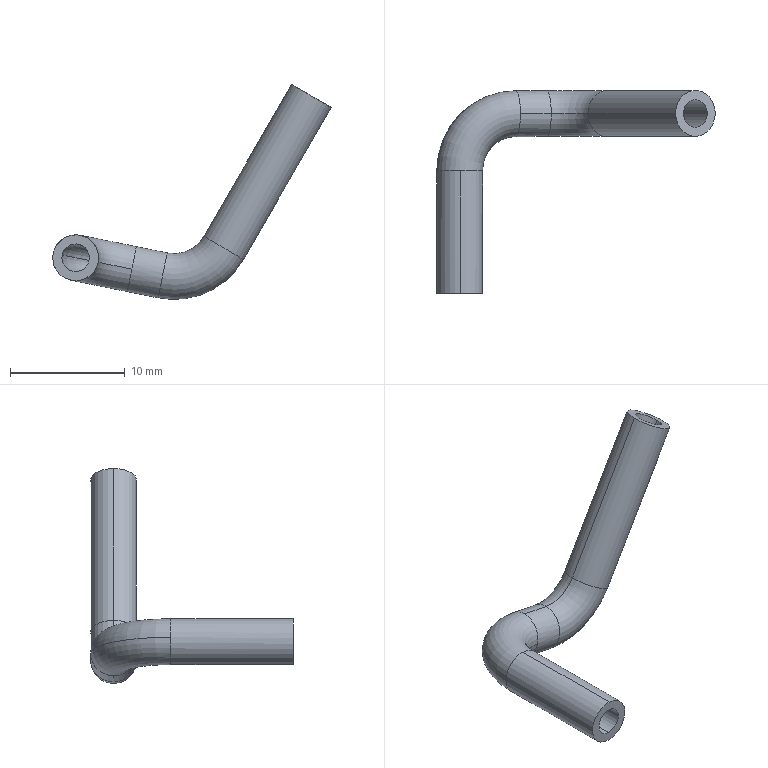Component | SolidWorks | WaterPipe7-1 | 1 solid | 22 faces | box 24.3 x 17.68 x 18.75 mm | volume 344 mm3 | cylinder 12 | torus 8 | plane 2 | commonest cylinder face diameters 2.4 x6 4 x6
build123d program:
from build123d import *

# Parameters (mm, degrees)
SCAN_THIN_FEATURE1_PROFILE_R   = 2
SCAN_THIN_FEATURE1_PROFILE_R_2 = 1.2


with BuildPart() as part:
    # Scan-Thin Feature1: sweep along a curve in space
    with BuildLine() as scan_thin_feature1_path:
        Line((10, -15, 0), (10, -4.322, 0))
        ThreePointArc((5.069, 0.6783, 0.8273), (8.556, -0.7862, 0.2423), (10, -4.322, 0))
        Line((5.069, 0.6783, 0.8273), (2.362, 0.6783, 1.281))
        ThreePointArc((-2.879, 0.6783, -1.299), (-0.6744, 0.6783, 0.836), (2.362, 0.6783, 1.281))
        Line((-2.879, 0.6783, -1.299), (-10.072, 0.6783, -14.805))
    # Scan-Thin Feature1 profile (on start of the path) → Scan-Thin Feature1 (sweep)
    with BuildSketch(Plane(origin=(10, -15, 0), x_dir=(0, 0, 1), z_dir=(0, 1, 0))):
        Circle(SCAN_THIN_FEATURE1_PROFILE_R)
        Circle(SCAN_THIN_FEATURE1_PROFILE_R_2, mode=Mode.SUBTRACT)
    sweep(path=scan_thin_feature1_path.line)


solid = part.part

# Placed as in the assembly
solid = solid.moved(Location((14.013, 32.882, 79.658), (180, -1.96, -180)))
STEP:
#1=COLOUR_RGB('',0.7922,0.8196,0.9333);
#2=FILL_AREA_STYLE_COLOUR('',#1);
#3=FILL_AREA_STYLE('',(#2));
#4=SURFACE_STYLE_FILL_AREA(#3);
#5=SURFACE_SIDE_STYLE('',(#4));
#6=SURFACE_STYLE_USAGE(.BOTH.,#5);
#7=PRESENTATION_STYLE_ASSIGNMENT((#6));
#8=CARTESIAN_POINT('',(0.4665,1.321,3.135));
#9=VERTEX_POINT('',#8);
#10=CARTESIAN_POINT('',(0.4476,1.321,3.043));
#11=VERTEX_POINT('',#10);
#12=CARTESIAN_POINT('',(0.457,1.321,3.089));
#13=DIRECTION('',(-0.98,-0.,0.1991));
#14=DIRECTION('',(-0.1991,0.,-0.98));
#15=AXIS2_PLACEMENT_3D('',#12,#13,#14);
#16=CIRCLE('',#15,0.04724);
#17=EDGE_CURVE('',#9,#11,#16,.T.);
#18=ORIENTED_EDGE('',*,*,#17,.T.);
#19=CARTESIAN_POINT('',(0.7076,1.321,3.16));
#20=VERTEX_POINT('',#19);
#21=CARTESIAN_POINT('',(0.4962,1.321,3.282));
#22=DIRECTION('',(0.,-1.,0.));
#23=DIRECTION('',(0.,0.,-1.));
#24=AXIS2_PLACEMENT_3D('',#21,#22,#23);
#25=CIRCLE('',#24,0.2441);
#26=EDGE_CURVE('',#11,#20,#25,.T.);
#27=ORIENTED_EDGE('',*,*,#26,.T.);
#28=CARTESIAN_POINT('',(0.6258,1.321,3.207));
#29=VERTEX_POINT('',#28);
#30=CARTESIAN_POINT('',(0.6667,1.321,3.183));
#31=DIRECTION('',(-0.5,-0.,-0.866));
#32=DIRECTION('',(-0.866,0.,0.5));
#33=AXIS2_PLACEMENT_3D('',#30,#31,#32);
#34=CIRCLE('',#33,0.04724);
#35=EDGE_CURVE('',#29,#20,#34,.T.);
#36=ORIENTED_EDGE('',*,*,#35,.F.);
#37=CARTESIAN_POINT('',(0.4962,1.321,3.282));
#38=DIRECTION('',(0.,-1.,0.));
#39=DIRECTION('',(0.,0.,-1.));
#40=AXIS2_PLACEMENT_3D('',#37,#38,#39);
#41=CIRCLE('',#40,0.1496);
#42=EDGE_CURVE('',#9,#29,#41,.T.);
#43=ORIENTED_EDGE('',*,*,#42,.F.);
#44=EDGE_LOOP('',(#18,#27,#36,#43));
#45=FACE_OUTER_BOUND('',#44,.T.);
#46=CARTESIAN_POINT('',(0.4962,1.321,3.282));
#47=DIRECTION('',(0.,-1.,0.));
#48=DIRECTION('',(0.03421,0.,0.9994));
#49=AXIS2_PLACEMENT_3D('',#46,#47,#48);
#50=TOROIDAL_SURFACE('',#49,0.1969,0.04724);
#51=ADVANCED_FACE('',(#45),#50,.F.);
#52=CARTESIAN_POINT('',(0.1598,1.124,3.197));
#53=VERTEX_POINT('',#52);
#54=CARTESIAN_POINT('',(0.1119,1.124,3.159));
#55=VERTEX_POINT('',#54);
#56=CARTESIAN_POINT('',(0.1582,1.124,3.15));
#57=DIRECTION('',(0.,-1.,0.));
#58=DIRECTION('',(-0.03421,0.,-0.9994));
#59=AXIS2_PLACEMENT_3D('',#56,#57,#58);
#60=CIRCLE('',#59,0.04724);
#61=EDGE_CURVE('',#53,#55,#60,.T.);
#62=ORIENTED_EDGE('',*,*,#61,.T.);
#63=CARTESIAN_POINT('',(0.3511,1.369,3.11));
#64=VERTEX_POINT('',#63);
#65=CARTESIAN_POINT('',(0.3511,1.124,3.11));
#66=DIRECTION('',(-0.1991,-0.,-0.98));
#67=DIRECTION('',(-0.98,0.,0.1991));
#68=AXIS2_PLACEMENT_3D('',#65,#66,#67);
#69=CIRCLE('',#68,0.2441);
#70=EDGE_CURVE('',#55,#64,#69,.T.);
#71=ORIENTED_EDGE('',*,*,#70,.T.);
#72=CARTESIAN_POINT('',(0.3605,1.321,3.157));
#73=VERTEX_POINT('',#72);
#74=CARTESIAN_POINT('',(0.3511,1.321,3.11));
#75=DIRECTION('',(-0.98,-0.,0.1991));
#76=DIRECTION('',(0.1991,0.,0.98));
#77=AXIS2_PLACEMENT_3D('',#74,#75,#76);
#78=CIRCLE('',#77,0.04724);
#79=EDGE_CURVE('',#73,#64,#78,.T.);
#80=ORIENTED_EDGE('',*,*,#79,.F.);
#81=CARTESIAN_POINT('',(0.3511,1.274,3.11));
#82=VERTEX_POINT('',#81);
#83=CARTESIAN_POINT('',(0.3511,1.321,3.11));
#84=DIRECTION('',(-0.98,-0.,0.1991));
#85=DIRECTION('',(0.1991,0.,0.98));
#86=AXIS2_PLACEMENT_3D('',#83,#84,#85);
#87=CIRCLE('',#86,0.04724);
#88=EDGE_CURVE('',#82,#73,#87,.T.);
#89=ORIENTED_EDGE('',*,*,#88,.F.);
#90=CARTESIAN_POINT('',(0.2045,1.124,3.14));
#91=VERTEX_POINT('',#90);
#92=CARTESIAN_POINT('',(0.3511,1.124,3.11));
#93=DIRECTION('',(-0.1991,-0.,-0.98));
#94=DIRECTION('',(-0.98,0.,0.1991));
#95=AXIS2_PLACEMENT_3D('',#92,#93,#94);
#96=CIRCLE('',#95,0.1496);
#97=EDGE_CURVE('',#91,#82,#96,.T.);
#98=ORIENTED_EDGE('',*,*,#97,.F.);
#99=CARTESIAN_POINT('',(0.1582,1.124,3.15));
#100=DIRECTION('',(0.,-1.,0.));
#101=DIRECTION('',(-0.03421,0.,-0.9994));
#102=AXIS2_PLACEMENT_3D('',#99,#100,#101);
#103=CIRCLE('',#102,0.04724);
#104=EDGE_CURVE('',#91,#53,#103,.T.);
#105=ORIENTED_EDGE('',*,*,#104,.T.);
#106=EDGE_LOOP('',(#62,#71,#80,#89,#98,#105));
#107=FACE_OUTER_BOUND('',#106,.T.);
#108=CARTESIAN_POINT('',(0.3511,1.124,3.11));
#109=DIRECTION('',(-0.1991,-0.,-0.98));
#110=DIRECTION('',(-0.98,-0.,0.1991));
#111=AXIS2_PLACEMENT_3D('',#108,#109,#110);
#112=TOROIDAL_SURFACE('',#111,0.1969,0.04724);
#113=ADVANCED_FACE('',(#107),#112,.F.);
#114=CARTESIAN_POINT('',(0.4414,1.321,3.012));
#115=VERTEX_POINT('',#114);
#116=CARTESIAN_POINT('',(0.4727,1.321,3.166));
#117=VERTEX_POINT('',#116);
#118=CARTESIAN_POINT('',(0.457,1.321,3.089));
#119=DIRECTION('',(-0.98,-0.,0.1991));
#120=DIRECTION('',(0.1991,0.,0.98));
#121=AXIS2_PLACEMENT_3D('',#118,#119,#120);
#122=CIRCLE('',#121,0.07874);
#123=EDGE_CURVE('',#115,#117,#122,.T.);
#124=ORIENTED_EDGE('',*,*,#123,.F.);
#125=CARTESIAN_POINT('',(0.7349,1.321,3.144));
#126=VERTEX_POINT('',#125);
#127=CARTESIAN_POINT('',(0.4962,1.321,3.282));
#128=DIRECTION('',(0.,-1.,0.));
#129=DIRECTION('',(0.,0.,-1.));
#130=AXIS2_PLACEMENT_3D('',#127,#128,#129);
#131=CIRCLE('',#130,0.2756);
#132=EDGE_CURVE('',#115,#126,#131,.T.);
#133=ORIENTED_EDGE('',*,*,#132,.T.);
#134=CARTESIAN_POINT('',(0.5985,1.321,3.223));
#135=VERTEX_POINT('',#134);
#136=CARTESIAN_POINT('',(0.6667,1.321,3.183));
#137=DIRECTION('',(-0.5,-0.,-0.866));
#138=DIRECTION('',(-0.866,0.,0.5));
#139=AXIS2_PLACEMENT_3D('',#136,#137,#138);
#140=CIRCLE('',#139,0.07874);
#141=EDGE_CURVE('',#126,#135,#140,.T.);
#142=ORIENTED_EDGE('',*,*,#141,.T.);
#143=CARTESIAN_POINT('',(0.4962,1.321,3.282));
#144=DIRECTION('',(0.,-1.,0.));
#145=DIRECTION('',(0.,0.,-1.));
#146=AXIS2_PLACEMENT_3D('',#143,#144,#145);
#147=CIRCLE('',#146,0.1181);
#148=EDGE_CURVE('',#117,#135,#147,.T.);
#149=ORIENTED_EDGE('',*,*,#148,.F.);
#150=EDGE_LOOP('',(#124,#133,#142,#149));
#151=FACE_OUTER_BOUND('',#150,.T.);
#152=CARTESIAN_POINT('',(0.4962,1.321,3.282));
#153=DIRECTION('',(0.,-1.,0.));
#154=DIRECTION('',(0.03421,0.,0.9994));
#155=AXIS2_PLACEMENT_3D('',#152,#153,#154);
#156=TOROIDAL_SURFACE('',#155,0.1969,0.07874);
#157=ADVANCED_FACE('',(#151),#156,.T.);
#158=CARTESIAN_POINT('',(0.08107,1.124,3.165));
#159=VERTEX_POINT('',#158);
#160=CARTESIAN_POINT('',(0.1555,1.124,3.071));
#161=VERTEX_POINT('',#160);
#162=CARTESIAN_POINT('',(0.1582,1.124,3.15));
#163=DIRECTION('',(0.,-1.,0.));
#164=DIRECTION('',(0.1991,0.,0.98));
#165=AXIS2_PLACEMENT_3D('',#162,#163,#164);
#166=CIRCLE('',#165,0.07874);
#167=EDGE_CURVE('',#159,#161,#166,.T.);
#168=ORIENTED_EDGE('',*,*,#167,.F.);
#169=CARTESIAN_POINT('',(0.3511,1.4,3.11));
#170=VERTEX_POINT('',#169);
#171=CARTESIAN_POINT('',(0.3511,1.124,3.11));
#172=DIRECTION('',(-0.1991,-0.,-0.98));
#173=DIRECTION('',(-0.98,0.,0.1991));
#174=AXIS2_PLACEMENT_3D('',#171,#172,#173);
#175=CIRCLE('',#174,0.2756);
#176=EDGE_CURVE('',#159,#170,#175,.T.);
#177=ORIENTED_EDGE('',*,*,#176,.T.);
#178=CARTESIAN_POINT('',(0.3355,1.321,3.033));
#179=VERTEX_POINT('',#178);
#180=CARTESIAN_POINT('',(0.3511,1.321,3.11));
#181=DIRECTION('',(-0.98,-0.,0.1991));
#182=DIRECTION('',(0.1991,0.,0.98));
#183=AXIS2_PLACEMENT_3D('',#180,#181,#182);
#184=CIRCLE('',#183,0.07874);
#185=EDGE_CURVE('',#170,#179,#184,.T.);
#186=ORIENTED_EDGE('',*,*,#185,.T.);
#187=CARTESIAN_POINT('',(0.3511,1.243,3.11));
#188=VERTEX_POINT('',#187);
#189=CARTESIAN_POINT('',(0.3511,1.321,3.11));
#190=DIRECTION('',(-0.98,-0.,0.1991));
#191=DIRECTION('',(0.1991,0.,0.98));
#192=AXIS2_PLACEMENT_3D('',#189,#190,#191);
#193=CIRCLE('',#192,0.07874);
#194=EDGE_CURVE('',#179,#188,#193,.T.);
#195=ORIENTED_EDGE('',*,*,#194,.T.);
#196=CARTESIAN_POINT('',(0.2354,1.124,3.134));
#197=VERTEX_POINT('',#196);
#198=CARTESIAN_POINT('',(0.3511,1.124,3.11));
#199=DIRECTION('',(-0.1991,-0.,-0.98));
#200=DIRECTION('',(-0.98,0.,0.1991));
#201=AXIS2_PLACEMENT_3D('',#198,#199,#200);
#202=CIRCLE('',#201,0.1181);
#203=EDGE_CURVE('',#197,#188,#202,.T.);
#204=ORIENTED_EDGE('',*,*,#203,.F.);
#205=CARTESIAN_POINT('',(0.1582,1.124,3.15));
#206=DIRECTION('',(0.,-1.,0.));
#207=DIRECTION('',(0.1991,0.,0.98));
#208=AXIS2_PLACEMENT_3D('',#205,#206,#207);
#209=CIRCLE('',#208,0.07874);
#210=EDGE_CURVE('',#161,#197,#209,.T.);
#211=ORIENTED_EDGE('',*,*,#210,.F.);
#212=EDGE_LOOP('',(#168,#177,#186,#195,#204,#211));
#213=FACE_OUTER_BOUND('',#212,.T.);
#214=CARTESIAN_POINT('',(0.3511,1.124,3.11));
#215=DIRECTION('',(-0.1991,-0.,-0.98));
#216=DIRECTION('',(-0.98,0.,0.1991));
#217=AXIS2_PLACEMENT_3D('',#214,#215,#216);
#218=TOROIDAL_SURFACE('',#217,0.1969,0.07874);
#219=ADVANCED_FACE('',(#213),#218,.T.);
#220=CARTESIAN_POINT('',(0.6667,1.321,3.183));
#221=DIRECTION('',(-0.5,-0.,-0.866));
#222=DIRECTION('',(-0.866,0.,0.5));
#223=AXIS2_PLACEMENT_3D('',#220,#221,#222);
#224=CIRCLE('',#223,0.04724);
#225=EDGE_CURVE('',#20,#29,#224,.T.);
#226=ORIENTED_EDGE('',*,*,#225,.T.);
#227=CARTESIAN_POINT('',(0.927,1.321,3.729));
#228=VERTEX_POINT('',#227);
#229=CARTESIAN_POINT('',(0.6258,1.321,3.207));
#230=DIRECTION('',(0.5,0.,0.866));
#231=VECTOR('',#230,39.37);
#232=LINE('',#229,#231);
#233=EDGE_CURVE('',#29,#228,#232,.T.);
#234=ORIENTED_EDGE('',*,*,#233,.T.);
#235=CARTESIAN_POINT('',(1.009,1.321,3.681));
#236=VERTEX_POINT('',#235);
#237=CARTESIAN_POINT('',(0.9679,1.321,3.705));
#238=DIRECTION('',(-0.5,-0.,-0.866));
#239=DIRECTION('',(-0.866,0.,0.5));
#240=AXIS2_PLACEMENT_3D('',#237,#238,#239);
#241=CIRCLE('',#240,0.04724);
#242=EDGE_CURVE('',#236,#228,#241,.T.);
#243=ORIENTED_EDGE('',*,*,#242,.F.);
#244=CARTESIAN_POINT('',(0.7076,1.321,3.16));
#245=DIRECTION('',(0.5,0.,0.866));
#246=VECTOR('',#245,39.37);
#247=LINE('',#244,#246);
#248=EDGE_CURVE('',#20,#236,#247,.T.);
#249=ORIENTED_EDGE('',*,*,#248,.F.);
#250=EDGE_LOOP('',(#226,#234,#243,#249));
#251=FACE_OUTER_BOUND('',#250,.T.);
#252=CARTESIAN_POINT('',(0.6667,1.321,3.183));
#253=DIRECTION('',(0.5,0.,0.866));
#254=DIRECTION('',(0.866,0.,-0.5));
#255=AXIS2_PLACEMENT_3D('',#252,#253,#254);
#256=CYLINDRICAL_SURFACE('',#255,0.04724);
#257=ADVANCED_FACE('',(#251),#256,.F.);
#258=CARTESIAN_POINT('',(0.3417,1.321,3.064));
#259=VERTEX_POINT('',#258);
#260=CARTESIAN_POINT('',(0.3511,1.321,3.11));
#261=DIRECTION('',(-0.98,-0.,0.1991));
#262=DIRECTION('',(0.1991,0.,0.98));
#263=AXIS2_PLACEMENT_3D('',#260,#261,#262);
#264=CIRCLE('',#263,0.04724);
#265=EDGE_CURVE('',#259,#82,#264,.T.);
#266=ORIENTED_EDGE('',*,*,#265,.T.);
#267=ORIENTED_EDGE('',*,*,#88,.T.);
#268=CARTESIAN_POINT('',(0.3605,1.321,3.157));
#269=DIRECTION('',(0.98,0.,-0.1991));
#270=VECTOR('',#269,39.37);
#271=LINE('',#268,#270);
#272=EDGE_CURVE('',#73,#9,#271,.T.);
#273=ORIENTED_EDGE('',*,*,#272,.T.);
#274=CARTESIAN_POINT('',(0.457,1.321,3.089));
#275=DIRECTION('',(-0.98,-0.,0.1991));
#276=DIRECTION('',(-0.1991,0.,-0.98));
#277=AXIS2_PLACEMENT_3D('',#274,#275,#276);
#278=CIRCLE('',#277,0.04724);
#279=EDGE_CURVE('',#11,#9,#278,.T.);
#280=ORIENTED_EDGE('',*,*,#279,.F.);
#281=CARTESIAN_POINT('',(0.3417,1.321,3.064));
#282=DIRECTION('',(0.98,0.,-0.1991));
#283=VECTOR('',#282,39.37);
#284=LINE('',#281,#283);
#285=EDGE_CURVE('',#259,#11,#284,.T.);
#286=ORIENTED_EDGE('',*,*,#285,.F.);
#287=EDGE_LOOP('',(#266,#267,#273,#280,#286));
#288=FACE_OUTER_BOUND('',#287,.T.);
#289=CARTESIAN_POINT('',(0.3511,1.321,3.11));
#290=DIRECTION('',(0.98,0.,-0.1991));
#291=DIRECTION('',(-0.1991,0.,-0.98));
#292=AXIS2_PLACEMENT_3D('',#289,#290,#291);
#293=CYLINDRICAL_SURFACE('',#292,0.04724);
#294=ADVANCED_FACE('',(#288),#293,.F.);
#295=CARTESIAN_POINT('',(0.1566,0.704,3.102));
#296=VERTEX_POINT('',#295);
#297=CARTESIAN_POINT('',(0.1598,0.704,3.197));
#298=VERTEX_POINT('',#297);
#299=CARTESIAN_POINT('',(0.1582,0.704,3.15));
#300=DIRECTION('',(0.,-1.,0.));
#301=DIRECTION('',(0.03421,0.,0.9994));
#302=AXIS2_PLACEMENT_3D('',#299,#300,#301);
#303=CIRCLE('',#302,0.04724);
#304=EDGE_CURVE('',#296,#298,#303,.T.);
#305=ORIENTED_EDGE('',*,*,#304,.T.);
#306=CARTESIAN_POINT('',(0.1598,0.704,3.197));
#307=DIRECTION('',(-0.,1.,-0.));
#308=VECTOR('',#307,39.37);
#309=LINE('',#306,#308);
#310=EDGE_CURVE('',#298,#53,#309,.T.);
#311=ORIENTED_EDGE('',*,*,#310,.T.);
#312=ORIENTED_EDGE('',*,*,#104,.F.);
#313=CARTESIAN_POINT('',(0.1566,1.124,3.102));
#314=VERTEX_POINT('',#313);
#315=CARTESIAN_POINT('',(0.1582,1.124,3.15));
#316=DIRECTION('',(0.,-1.,0.));
#317=DIRECTION('',(-0.03421,0.,-0.9994));
#318=AXIS2_PLACEMENT_3D('',#315,#316,#317);
#319=CIRCLE('',#318,0.04724);
#320=EDGE_CURVE('',#314,#91,#319,.T.);
#321=ORIENTED_EDGE('',*,*,#320,.F.);
#322=CARTESIAN_POINT('',(0.1566,0.704,3.102));
#323=DIRECTION('',(-0.,1.,-0.));
#324=VECTOR('',#323,39.37);
#325=LINE('',#322,#324);
#326=EDGE_CURVE('',#296,#314,#325,.T.);
#327=ORIENTED_EDGE('',*,*,#326,.F.);
#328=EDGE_LOOP('',(#305,#311,#312,#321,#327));
#329=FACE_OUTER_BOUND('',#328,.T.);
#330=CARTESIAN_POINT('',(0.1582,0.704,3.15));
#331=DIRECTION('',(-0.,1.,-0.));
#332=DIRECTION('',(-0.03421,0.,-0.9994));
#333=AXIS2_PLACEMENT_3D('',#330,#331,#332);
#334=CYLINDRICAL_SURFACE('',#333,0.04724);
#335=ADVANCED_FACE('',(#329),#334,.F.);
#336=CARTESIAN_POINT('',(0.6667,1.321,3.183));
#337=DIRECTION('',(-0.5,-0.,-0.866));
#338=DIRECTION('',(-0.866,0.,0.5));
#339=AXIS2_PLACEMENT_3D('',#336,#337,#338);
#340=CIRCLE('',#339,0.07874);
#341=EDGE_CURVE('',#135,#126,#340,.T.);
#342=ORIENTED_EDGE('',*,*,#341,.F.);
#343=CARTESIAN_POINT('',(0.8997,1.321,3.744));
#344=VERTEX_POINT('',#343);
#345=CARTESIAN_POINT('',(0.5985,1.321,3.223));
#346=DIRECTION('',(0.5,0.,0.866));
#347=VECTOR('',#346,39.37);
#348=LINE('',#345,#347);
#349=EDGE_CURVE('',#135,#344,#348,.T.);
#350=ORIENTED_EDGE('',*,*,#349,.T.);
#351=CARTESIAN_POINT('',(1.036,1.321,3.666));
#352=VERTEX_POINT('',#351);
#353=CARTESIAN_POINT('',(0.9679,1.321,3.705));
#354=DIRECTION('',(-0.5,-0.,-0.866));
#355=DIRECTION('',(-0.866,0.,0.5));
#356=AXIS2_PLACEMENT_3D('',#353,#354,#355);
#357=CIRCLE('',#356,0.07874);
#358=EDGE_CURVE('',#344,#352,#357,.T.);
#359=ORIENTED_EDGE('',*,*,#358,.T.);
#360=CARTESIAN_POINT('',(0.7349,1.321,3.144));
#361=DIRECTION('',(0.5,0.,0.866));
#362=VECTOR('',#361,39.37);
#363=LINE('',#360,#362);
#364=EDGE_CURVE('',#126,#352,#363,.T.);
#365=ORIENTED_EDGE('',*,*,#364,.F.);
#366=EDGE_LOOP('',(#342,#350,#359,#365));
#367=FACE_OUTER_BOUND('',#366,.T.);
#368=CARTESIAN_POINT('',(0.6667,1.321,3.183));
#369=DIRECTION('',(0.5,0.,0.866));
#370=DIRECTION('',(0.866,0.,-0.5));
#371=AXIS2_PLACEMENT_3D('',#368,#369,#370);
#372=CYLINDRICAL_SURFACE('',#371,0.07874);
#373=ADVANCED_FACE('',(#367),#372,.T.);
#374=CARTESIAN_POINT('',(0.3668,1.321,3.188));
#375=VERTEX_POINT('',#374);
#376=CARTESIAN_POINT('',(0.3511,1.321,3.11));
#377=DIRECTION('',(-0.98,-0.,0.1991));
#378=DIRECTION('',(0.1991,0.,0.98));
#379=AXIS2_PLACEMENT_3D('',#376,#377,#378);
#380=CIRCLE('',#379,0.07874);
#381=EDGE_CURVE('',#375,#170,#380,.T.);
#382=ORIENTED_EDGE('',*,*,#381,.F.);
#383=CARTESIAN_POINT('',(0.3668,1.321,3.188));
#384=DIRECTION('',(0.98,0.,-0.1991));
#385=VECTOR('',#384,39.37);
#386=LINE('',#383,#385);
#387=EDGE_CURVE('',#375,#117,#386,.T.);
#388=ORIENTED_EDGE('',*,*,#387,.T.);
#389=CARTESIAN_POINT('',(0.457,1.321,3.089));
#390=DIRECTION('',(-0.98,-0.,0.1991));
#391=DIRECTION('',(0.1991,0.,0.98));
#392=AXIS2_PLACEMENT_3D('',#389,#390,#391);
#393=CIRCLE('',#392,0.07874);
#394=EDGE_CURVE('',#117,#115,#393,.T.);
#395=ORIENTED_EDGE('',*,*,#394,.T.);
#396=CARTESIAN_POINT('',(0.3355,1.321,3.033));
#397=DIRECTION('',(0.98,0.,-0.1991));
#398=VECTOR('',#397,39.37);
#399=LINE('',#396,#398);
#400=EDGE_CURVE('',#179,#115,#399,.T.);
#401=ORIENTED_EDGE('',*,*,#400,.F.);
#402=ORIENTED_EDGE('',*,*,#185,.F.);
#403=EDGE_LOOP('',(#382,#388,#395,#401,#402));
#404=FACE_OUTER_BOUND('',#403,.T.);
#405=CARTESIAN_POINT('',(0.3511,1.321,3.11));
#406=DIRECTION('',(0.98,0.,-0.1991));
#407=DIRECTION('',(-0.1991,0.,-0.98));
#408=AXIS2_PLACEMENT_3D('',#405,#406,#407);
#409=CYLINDRICAL_SURFACE('',#408,0.07874);
#410=ADVANCED_FACE('',(#404),#409,.T.);
#411=CARTESIAN_POINT('',(0.1609,0.704,3.228));
#412=VERTEX_POINT('',#411);
#413=CARTESIAN_POINT('',(0.1555,0.704,3.071));
#414=VERTEX_POINT('',#413);
#415=CARTESIAN_POINT('',(0.1582,0.704,3.15));
#416=DIRECTION('',(0.,-1.,0.));
#417=DIRECTION('',(0.1991,0.,0.98));
#418=AXIS2_PLACEMENT_3D('',#415,#416,#417);
#419=CIRCLE('',#418,0.07874);
#420=EDGE_CURVE('',#412,#414,#419,.T.);
#421=ORIENTED_EDGE('',*,*,#420,.F.);
#422=CARTESIAN_POINT('',(0.1609,1.124,3.228));
#423=VERTEX_POINT('',#422);
#424=CARTESIAN_POINT('',(0.1609,0.704,3.228));
#425=DIRECTION('',(-0.,1.,-0.));
#426=VECTOR('',#425,39.37);
#427=LINE('',#424,#426);
#428=EDGE_CURVE('',#412,#423,#427,.T.);
#429=ORIENTED_EDGE('',*,*,#428,.T.);
#430=CARTESIAN_POINT('',(0.1582,1.124,3.15));
#431=DIRECTION('',(0.,-1.,0.));
#432=DIRECTION('',(0.1991,0.,0.98));
#433=AXIS2_PLACEMENT_3D('',#430,#431,#432);
#434=CIRCLE('',#433,0.07874);
#435=EDGE_CURVE('',#423,#159,#434,.T.);
#436=ORIENTED_EDGE('',*,*,#435,.T.);
#437=ORIENTED_EDGE('',*,*,#167,.T.);
#438=CARTESIAN_POINT('',(0.1555,0.704,3.071));
#439=DIRECTION('',(-0.,1.,-0.));
#440=VECTOR('',#439,39.37);
#441=LINE('',#438,#440);
#442=EDGE_CURVE('',#414,#161,#441,.T.);
#443=ORIENTED_EDGE('',*,*,#442,.F.);
#444=EDGE_LOOP('',(#421,#429,#436,#437,#443));
#445=FACE_OUTER_BOUND('',#444,.T.);
#446=CARTESIAN_POINT('',(0.1582,0.704,3.15));
#447=DIRECTION('',(-0.,1.,-0.));
#448=DIRECTION('',(-0.03421,0.,-0.9994));
#449=AXIS2_PLACEMENT_3D('',#446,#447,#448);
#450=CYLINDRICAL_SURFACE('',#449,0.07874);
#451=ADVANCED_FACE('',(#445),#450,.T.);
#452=ORIENTED_EDGE('',*,*,#349,.F.);
#453=ORIENTED_EDGE('',*,*,#141,.F.);
#454=ORIENTED_EDGE('',*,*,#364,.T.);
#455=CARTESIAN_POINT('',(0.9679,1.321,3.705));
#456=DIRECTION('',(-0.5,-0.,-0.866));
#457=DIRECTION('',(-0.866,0.,0.5));
#458=AXIS2_PLACEMENT_3D('',#455,#456,#457);
#459=CIRCLE('',#458,0.07874);
#460=EDGE_CURVE('',#352,#344,#459,.T.);
#461=ORIENTED_EDGE('',*,*,#460,.T.);
#462=EDGE_LOOP('',(#452,#453,#454,#461));
#463=FACE_OUTER_BOUND('',#462,.T.);
#464=CARTESIAN_POINT('',(0.6667,1.321,3.183));
#465=DIRECTION('',(0.5,0.,0.866));
#466=DIRECTION('',(0.866,0.,-0.5));
#467=AXIS2_PLACEMENT_3D('',#464,#465,#466);
#468=CYLINDRICAL_SURFACE('',#467,0.07874);
#469=ADVANCED_FACE('',(#463),#468,.T.);
#470=ORIENTED_EDGE('',*,*,#132,.F.);
#471=ORIENTED_EDGE('',*,*,#394,.F.);
#472=ORIENTED_EDGE('',*,*,#148,.T.);
#473=ORIENTED_EDGE('',*,*,#341,.T.);
#474=EDGE_LOOP('',(#470,#471,#472,#473));
#475=FACE_OUTER_BOUND('',#474,.T.);
#476=CARTESIAN_POINT('',(0.4962,1.321,3.282));
#477=DIRECTION('',(0.,-1.,0.));
#478=DIRECTION('',(0.03421,0.,0.9994));
#479=AXIS2_PLACEMENT_3D('',#476,#477,#478);
#480=TOROIDAL_SURFACE('',#479,0.1969,0.07874);
#481=ADVANCED_FACE('',(#475),#480,.T.);
#482=ORIENTED_EDGE('',*,*,#387,.F.);
#483=CARTESIAN_POINT('',(0.3511,1.321,3.11));
#484=DIRECTION('',(-0.98,-0.,0.1991));
#485=DIRECTION('',(0.1991,0.,0.98));
#486=AXIS2_PLACEMENT_3D('',#483,#484,#485);
#487=CIRCLE('',#486,0.07874);
#488=EDGE_CURVE('',#188,#375,#487,.T.);
#489=ORIENTED_EDGE('',*,*,#488,.F.);
#490=ORIENTED_EDGE('',*,*,#194,.F.);
#491=ORIENTED_EDGE('',*,*,#400,.T.);
#492=ORIENTED_EDGE('',*,*,#123,.T.);
#493=EDGE_LOOP('',(#482,#489,#490,#491,#492));
#494=FACE_OUTER_BOUND('',#493,.T.);
#495=CARTESIAN_POINT('',(0.3511,1.321,3.11));
#496=DIRECTION('',(0.98,0.,-0.1991));
#497=DIRECTION('',(-0.1991,0.,-0.98));
#498=AXIS2_PLACEMENT_3D('',#495,#496,#497);
#499=CYLINDRICAL_SURFACE('',#498,0.07874);
#500=ADVANCED_FACE('',(#494),#499,.T.);
#501=ORIENTED_EDGE('',*,*,#176,.F.);
#502=ORIENTED_EDGE('',*,*,#435,.F.);
#503=CARTESIAN_POINT('',(0.1582,1.124,3.15));
#504=DIRECTION('',(0.,-1.,0.));
#505=DIRECTION('',(0.1991,0.,0.98));
#506=AXIS2_PLACEMENT_3D('',#503,#504,#505);
#507=CIRCLE('',#506,0.07874);
#508=EDGE_CURVE('',#197,#423,#507,.T.);
#509=ORIENTED_EDGE('',*,*,#508,.F.);
#510=ORIENTED_EDGE('',*,*,#203,.T.);
#511=ORIENTED_EDGE('',*,*,#488,.T.);
#512=ORIENTED_EDGE('',*,*,#381,.T.);
#513=EDGE_LOOP('',(#501,#502,#509,#510,#511,#512));
#514=FACE_OUTER_BOUND('',#513,.T.);
#515=CARTESIAN_POINT('',(0.3511,1.124,3.11));
#516=DIRECTION('',(-0.1991,-0.,-0.98));
#517=DIRECTION('',(-0.98,0.,0.1991));
#518=AXIS2_PLACEMENT_3D('',#515,#516,#517);
#519=TOROIDAL_SURFACE('',#518,0.1969,0.07874);
#520=ADVANCED_FACE('',(#514),#519,.T.);
#521=ORIENTED_EDGE('',*,*,#428,.F.);
#522=CARTESIAN_POINT('',(0.1582,0.704,3.15));
#523=DIRECTION('',(0.,-1.,0.));
#524=DIRECTION('',(0.1991,0.,0.98));
#525=AXIS2_PLACEMENT_3D('',#522,#523,#524);
#526=CIRCLE('',#525,0.07874);
#527=EDGE_CURVE('',#414,#412,#526,.T.);
#528=ORIENTED_EDGE('',*,*,#527,.F.);
#529=ORIENTED_EDGE('',*,*,#442,.T.);
#530=ORIENTED_EDGE('',*,*,#210,.T.);
#531=ORIENTED_EDGE('',*,*,#508,.T.);
#532=EDGE_LOOP('',(#521,#528,#529,#530,#531));
#533=FACE_OUTER_BOUND('',#532,.T.);
#534=CARTESIAN_POINT('',(0.1582,0.704,3.15));
#535=DIRECTION('',(-0.,1.,-0.));
#536=DIRECTION('',(-0.03421,0.,-0.9994));
#537=AXIS2_PLACEMENT_3D('',#534,#535,#536);
#538=CYLINDRICAL_SURFACE('',#537,0.07874);
#539=ADVANCED_FACE('',(#533),#538,.T.);
#540=ORIENTED_EDGE('',*,*,#242,.T.);
#541=CARTESIAN_POINT('',(0.9679,1.321,3.705));
#542=DIRECTION('',(-0.5,-0.,-0.866));
#543=DIRECTION('',(-0.866,0.,0.5));
#544=AXIS2_PLACEMENT_3D('',#541,#542,#543);
#545=CIRCLE('',#544,0.04724);
#546=EDGE_CURVE('',#228,#236,#545,.T.);
#547=ORIENTED_EDGE('',*,*,#546,.T.);
#548=EDGE_LOOP('',(#540,#547));
#549=FACE_BOUND('',#548,.T.);
#550=ORIENTED_EDGE('',*,*,#460,.F.);
#551=ORIENTED_EDGE('',*,*,#358,.F.);
#552=EDGE_LOOP('',(#550,#551));
#553=FACE_OUTER_BOUND('',#552,.T.);
#554=CARTESIAN_POINT('',(0.9679,1.321,3.705));
#555=DIRECTION('',(-0.5,-0.,-0.866));
#556=DIRECTION('',(-0.866,0.,0.5));
#557=AXIS2_PLACEMENT_3D('',#554,#555,#556);
#558=PLANE('',#557);
#559=ADVANCED_FACE('',(#549,#553),#558,.F.);
#560=ORIENTED_EDGE('',*,*,#304,.F.);
#561=CARTESIAN_POINT('',(0.1582,0.704,3.15));
#562=DIRECTION('',(0.,-1.,0.));
#563=DIRECTION('',(0.03421,0.,0.9994));
#564=AXIS2_PLACEMENT_3D('',#561,#562,#563);
#565=CIRCLE('',#564,0.04724);
#566=EDGE_CURVE('',#298,#296,#565,.T.);
#567=ORIENTED_EDGE('',*,*,#566,.F.);
#568=EDGE_LOOP('',(#560,#567));
#569=FACE_BOUND('',#568,.T.);
#570=ORIENTED_EDGE('',*,*,#527,.T.);
#571=ORIENTED_EDGE('',*,*,#420,.T.);
#572=EDGE_LOOP('',(#570,#571));
#573=FACE_OUTER_BOUND('',#572,.T.);
#574=CARTESIAN_POINT('',(0.1582,0.704,3.15));
#575=DIRECTION('',(0.,-1.,0.));
#576=DIRECTION('',(0.1991,0.,0.98));
#577=AXIS2_PLACEMENT_3D('',#574,#575,#576);
#578=PLANE('',#577);
#579=ADVANCED_FACE('',(#569,#573),#578,.T.);
#580=ORIENTED_EDGE('',*,*,#233,.F.);
#581=ORIENTED_EDGE('',*,*,#35,.T.);
#582=ORIENTED_EDGE('',*,*,#248,.T.);
#583=ORIENTED_EDGE('',*,*,#546,.F.);
#584=EDGE_LOOP('',(#580,#581,#582,#583));
#585=FACE_OUTER_BOUND('',#584,.T.);
#586=CARTESIAN_POINT('',(0.6667,1.321,3.183));
#587=DIRECTION('',(0.5,0.,0.866));
#588=DIRECTION('',(0.866,0.,-0.5));
#589=AXIS2_PLACEMENT_3D('',#586,#587,#588);
#590=CYLINDRICAL_SURFACE('',#589,0.04724);
#591=ADVANCED_FACE('',(#585),#590,.F.);
#592=ORIENTED_EDGE('',*,*,#26,.F.);
#593=ORIENTED_EDGE('',*,*,#279,.T.);
#594=ORIENTED_EDGE('',*,*,#42,.T.);
#595=ORIENTED_EDGE('',*,*,#225,.F.);
#596=EDGE_LOOP('',(#592,#593,#594,#595));
#597=FACE_OUTER_BOUND('',#596,.T.);
#598=CARTESIAN_POINT('',(0.4962,1.321,3.282));
#599=DIRECTION('',(0.,-1.,0.));
#600=DIRECTION('',(0.03421,0.,0.9994));
#601=AXIS2_PLACEMENT_3D('',#598,#599,#600);
#602=TOROIDAL_SURFACE('',#601,0.1969,0.04724);
#603=ADVANCED_FACE('',(#597),#602,.F.);
#604=ORIENTED_EDGE('',*,*,#272,.F.);
#605=ORIENTED_EDGE('',*,*,#79,.T.);
#606=CARTESIAN_POINT('',(0.3511,1.321,3.11));
#607=DIRECTION('',(-0.98,-0.,0.1991));
#608=DIRECTION('',(0.1991,0.,0.98));
#609=AXIS2_PLACEMENT_3D('',#606,#607,#608);
#610=CIRCLE('',#609,0.04724);
#611=EDGE_CURVE('',#64,#259,#610,.T.);
#612=ORIENTED_EDGE('',*,*,#611,.T.);
#613=ORIENTED_EDGE('',*,*,#285,.T.);
#614=ORIENTED_EDGE('',*,*,#17,.F.);
#615=EDGE_LOOP('',(#604,#605,#612,#613,#614));
#616=FACE_OUTER_BOUND('',#615,.T.);
#617=CARTESIAN_POINT('',(0.3511,1.321,3.11));
#618=DIRECTION('',(0.98,0.,-0.1991));
#619=DIRECTION('',(-0.1991,0.,-0.98));
#620=AXIS2_PLACEMENT_3D('',#617,#618,#619);
#621=CYLINDRICAL_SURFACE('',#620,0.04724);
#622=ADVANCED_FACE('',(#616),#621,.F.);
#623=ORIENTED_EDGE('',*,*,#70,.F.);
#624=CARTESIAN_POINT('',(0.1582,1.124,3.15));
#625=DIRECTION('',(0.,-1.,0.));
#626=DIRECTION('',(-0.03421,0.,-0.9994));
#627=AXIS2_PLACEMENT_3D('',#624,#625,#626);
#628=CIRCLE('',#627,0.04724);
#629=EDGE_CURVE('',#55,#314,#628,.T.);
#630=ORIENTED_EDGE('',*,*,#629,.T.);
#631=ORIENTED_EDGE('',*,*,#320,.T.);
#632=ORIENTED_EDGE('',*,*,#97,.T.);
#633=ORIENTED_EDGE('',*,*,#265,.F.);
#634=ORIENTED_EDGE('',*,*,#611,.F.);
#635=EDGE_LOOP('',(#623,#630,#631,#632,#633,#634));
#636=FACE_OUTER_BOUND('',#635,.T.);
#637=CARTESIAN_POINT('',(0.3511,1.124,3.11));
#638=DIRECTION('',(-0.1991,-0.,-0.98));
#639=DIRECTION('',(-0.98,-0.,0.1991));
#640=AXIS2_PLACEMENT_3D('',#637,#638,#639);
#641=TOROIDAL_SURFACE('',#640,0.1969,0.04724);
#642=ADVANCED_FACE('',(#636),#641,.F.);
#643=ORIENTED_EDGE('',*,*,#310,.F.);
#644=ORIENTED_EDGE('',*,*,#566,.T.);
#645=ORIENTED_EDGE('',*,*,#326,.T.);
#646=ORIENTED_EDGE('',*,*,#629,.F.);
#647=ORIENTED_EDGE('',*,*,#61,.F.);
#648=EDGE_LOOP('',(#643,#644,#645,#646,#647));
#649=FACE_OUTER_BOUND('',#648,.T.);
#650=CARTESIAN_POINT('',(0.1582,0.704,3.15));
#651=DIRECTION('',(-0.,1.,-0.));
#652=DIRECTION('',(-0.03421,0.,-0.9994));
#653=AXIS2_PLACEMENT_3D('',#650,#651,#652);
#654=CYLINDRICAL_SURFACE('',#653,0.04724);
#655=ADVANCED_FACE('',(#649),#654,.F.);
#656=CLOSED_SHELL('',(#51,#113,#157,#219,#257,#294,#335,#373,#410,#451,#469,#481,#500,#520,#539,#559,#579,#591,#603,#622,#642,#655));
#657=MANIFOLD_SOLID_BREP('',#656);
#658=STYLED_ITEM('',(#7),#657);
#659=(LENGTH_UNIT()NAMED_UNIT(*)SI_UNIT($,.METRE.));
#660=LENGTH_MEASURE_WITH_UNIT(LENGTH_MEASURE(0.0254),#659);
#661=DIMENSIONAL_EXPONENTS(1.,0.,0.,0.,0.,0.,0.);
#662=(CONVERSION_BASED_UNIT('',#660)LENGTH_UNIT()NAMED_UNIT(#661));
#663=UNCERTAINTY_MEASURE_WITH_UNIT(LENGTH_MEASURE(0.00001),#662,'','');
#664=(NAMED_UNIT(*)PLANE_ANGLE_UNIT()SI_UNIT($,.RADIAN.));
#665=(NAMED_UNIT(*)SI_UNIT($,.STERADIAN.)SOLID_ANGLE_UNIT());
#666=(GEOMETRIC_REPRESENTATION_CONTEXT(3)GLOBAL_UNCERTAINTY_ASSIGNED_CONTEXT((#663))GLOBAL_UNIT_ASSIGNED_CONTEXT((#662,#664,#665))REPRESENTATION_CONTEXT('',''));
#667=MECHANICAL_DESIGN_GEOMETRIC_PRESENTATION_REPRESENTATION('',(#658),#666);
#668=PRESENTATION_LAYER_ASSIGNMENT('','',(#658));
#669=CARTESIAN_POINT('',(0.,0.,0.));
#670=DIRECTION('',(0.,0.,1.));
#671=DIRECTION('',(1.,0.,0.));
#672=AXIS2_PLACEMENT_3D('',#669,#670,#671);
#673=(LENGTH_UNIT()NAMED_UNIT(*)SI_UNIT($,.METRE.));
#674=LENGTH_MEASURE_WITH_UNIT(LENGTH_MEASURE(0.0254),#673);
#675=DIMENSIONAL_EXPONENTS(1.,0.,0.,0.,0.,0.,0.);
#676=(CONVERSION_BASED_UNIT('',#674)LENGTH_UNIT()NAMED_UNIT(#675));
#677=UNCERTAINTY_MEASURE_WITH_UNIT(LENGTH_MEASURE(0.00001),#676,'','');
#678=(NAMED_UNIT(*)PLANE_ANGLE_UNIT()SI_UNIT($,.RADIAN.));
#679=(NAMED_UNIT(*)SI_UNIT($,.STERADIAN.)SOLID_ANGLE_UNIT());
#680=(GEOMETRIC_REPRESENTATION_CONTEXT(3)GLOBAL_UNCERTAINTY_ASSIGNED_CONTEXT((#677))GLOBAL_UNIT_ASSIGNED_CONTEXT((#676,#678,#679))REPRESENTATION_CONTEXT('',''));
#681=ADVANCED_BREP_SHAPE_REPRESENTATION('',(#657,#672),#680);